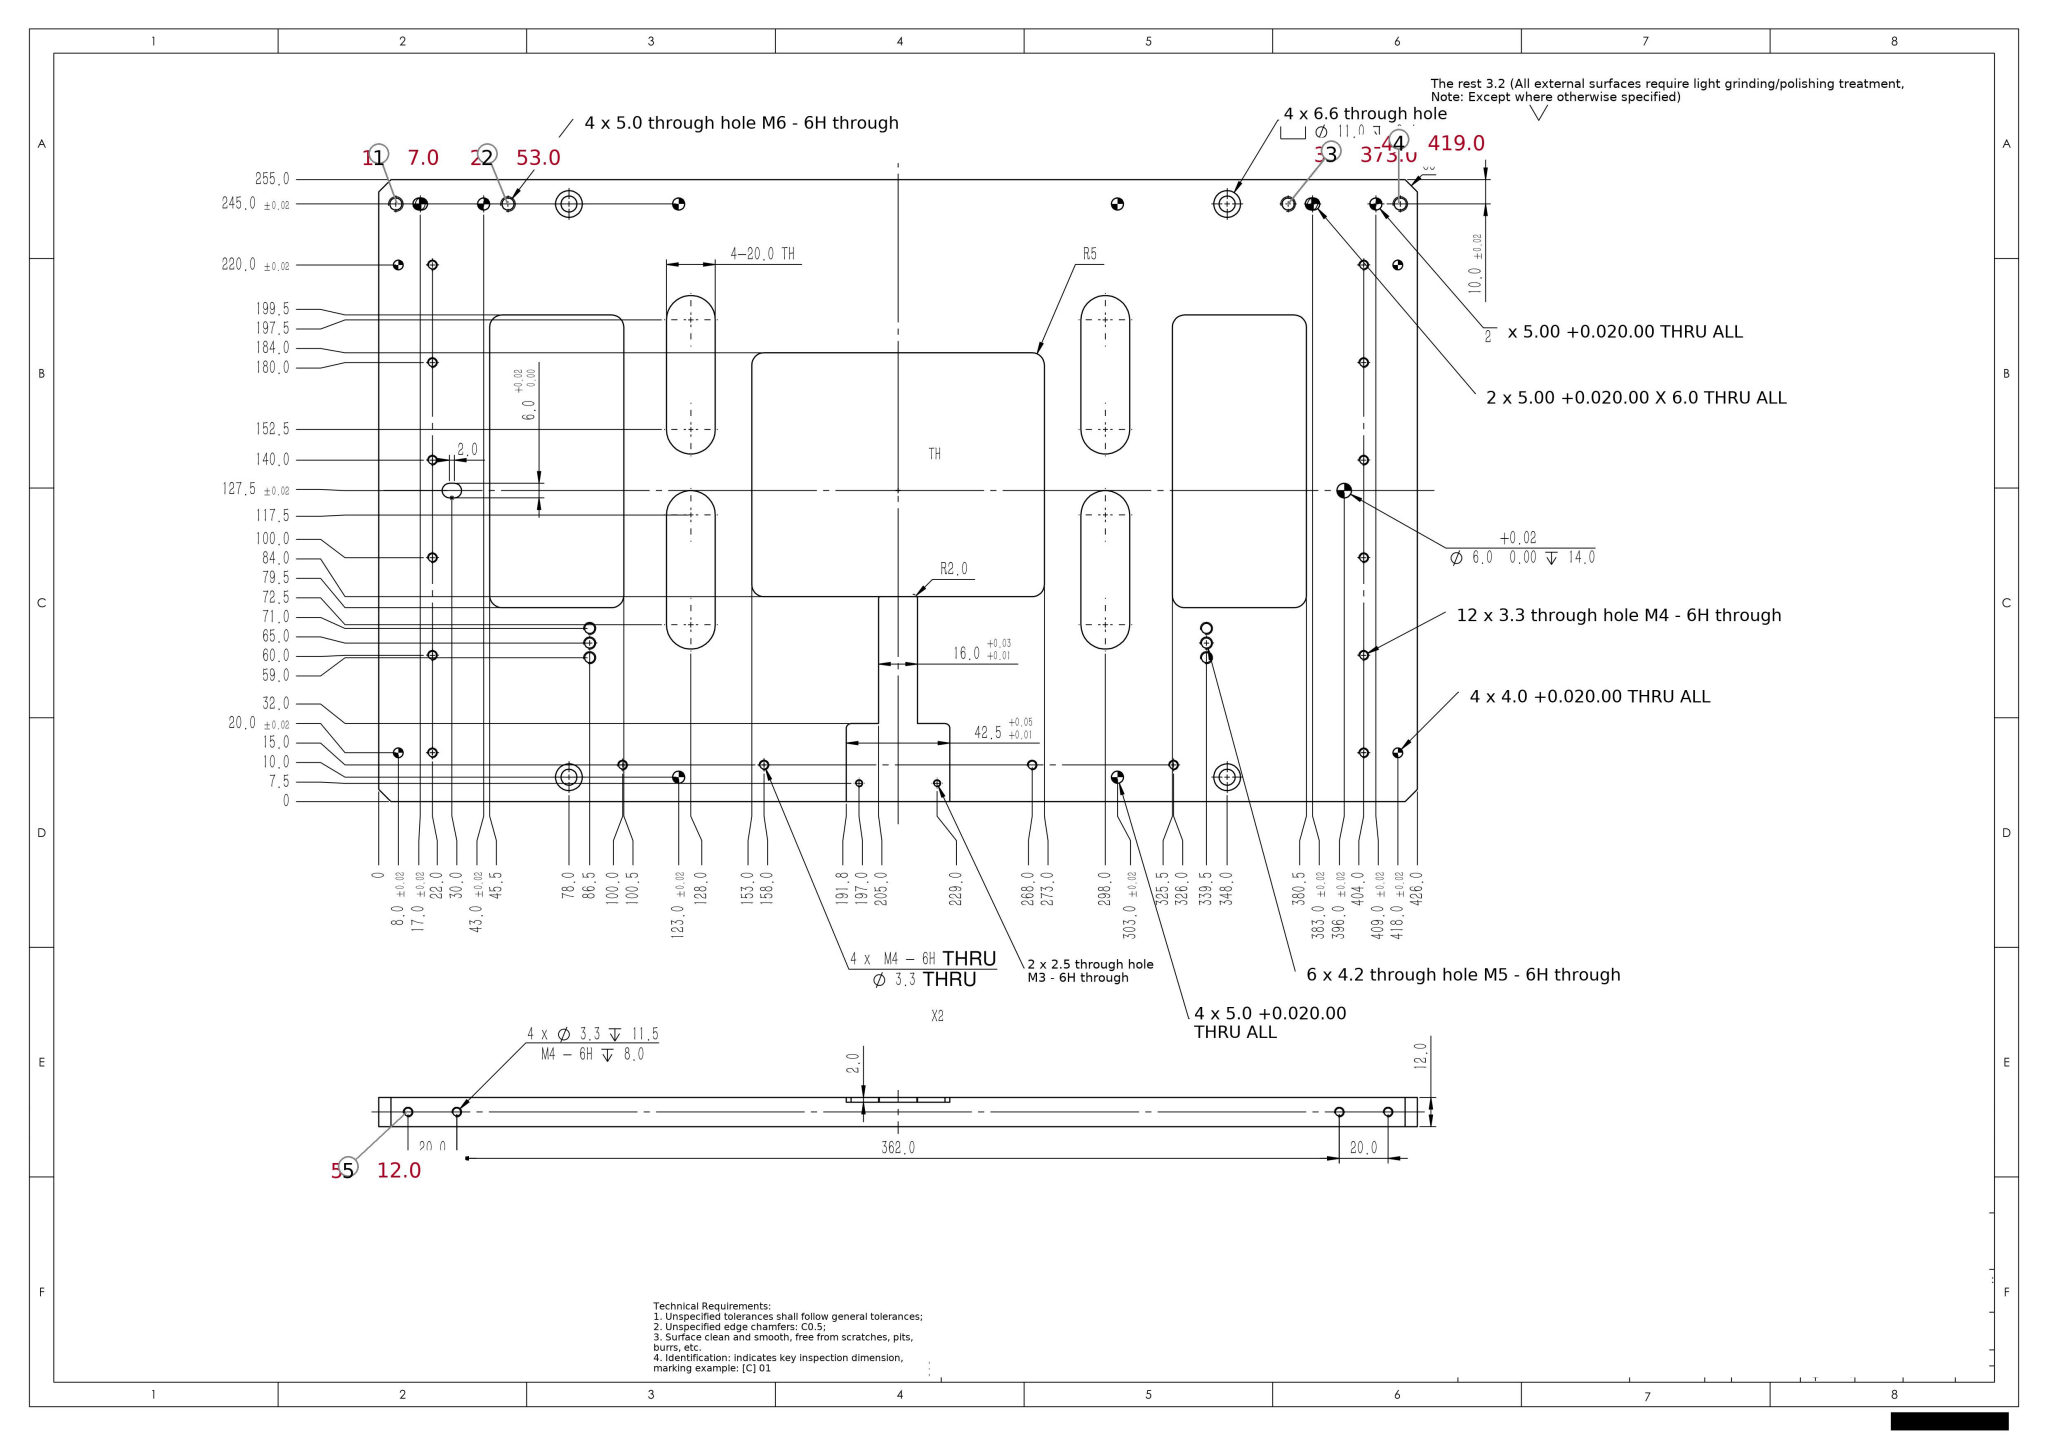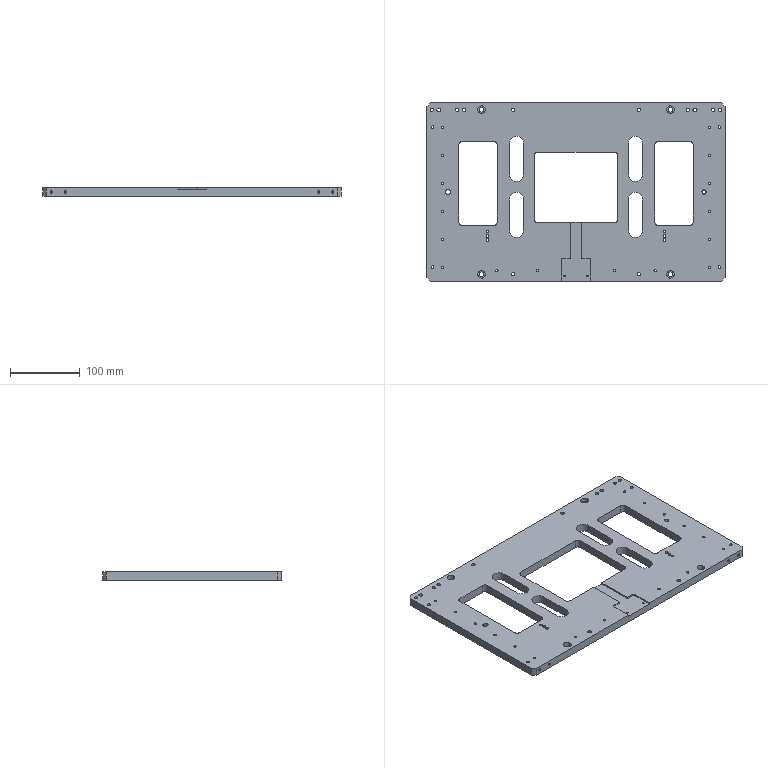Part | SolidWorks | mm | 1 solid | 190 faces | box 426 x 255 x 12 mm | volume 927958 mm3 | cylinder 135 | plane 47 | cone 8 | commonest cylinder face diameters 3.3 x40 5 x26 4 x12 4.2 x12 10 x12 11 x8 6.6 x8 20 x8